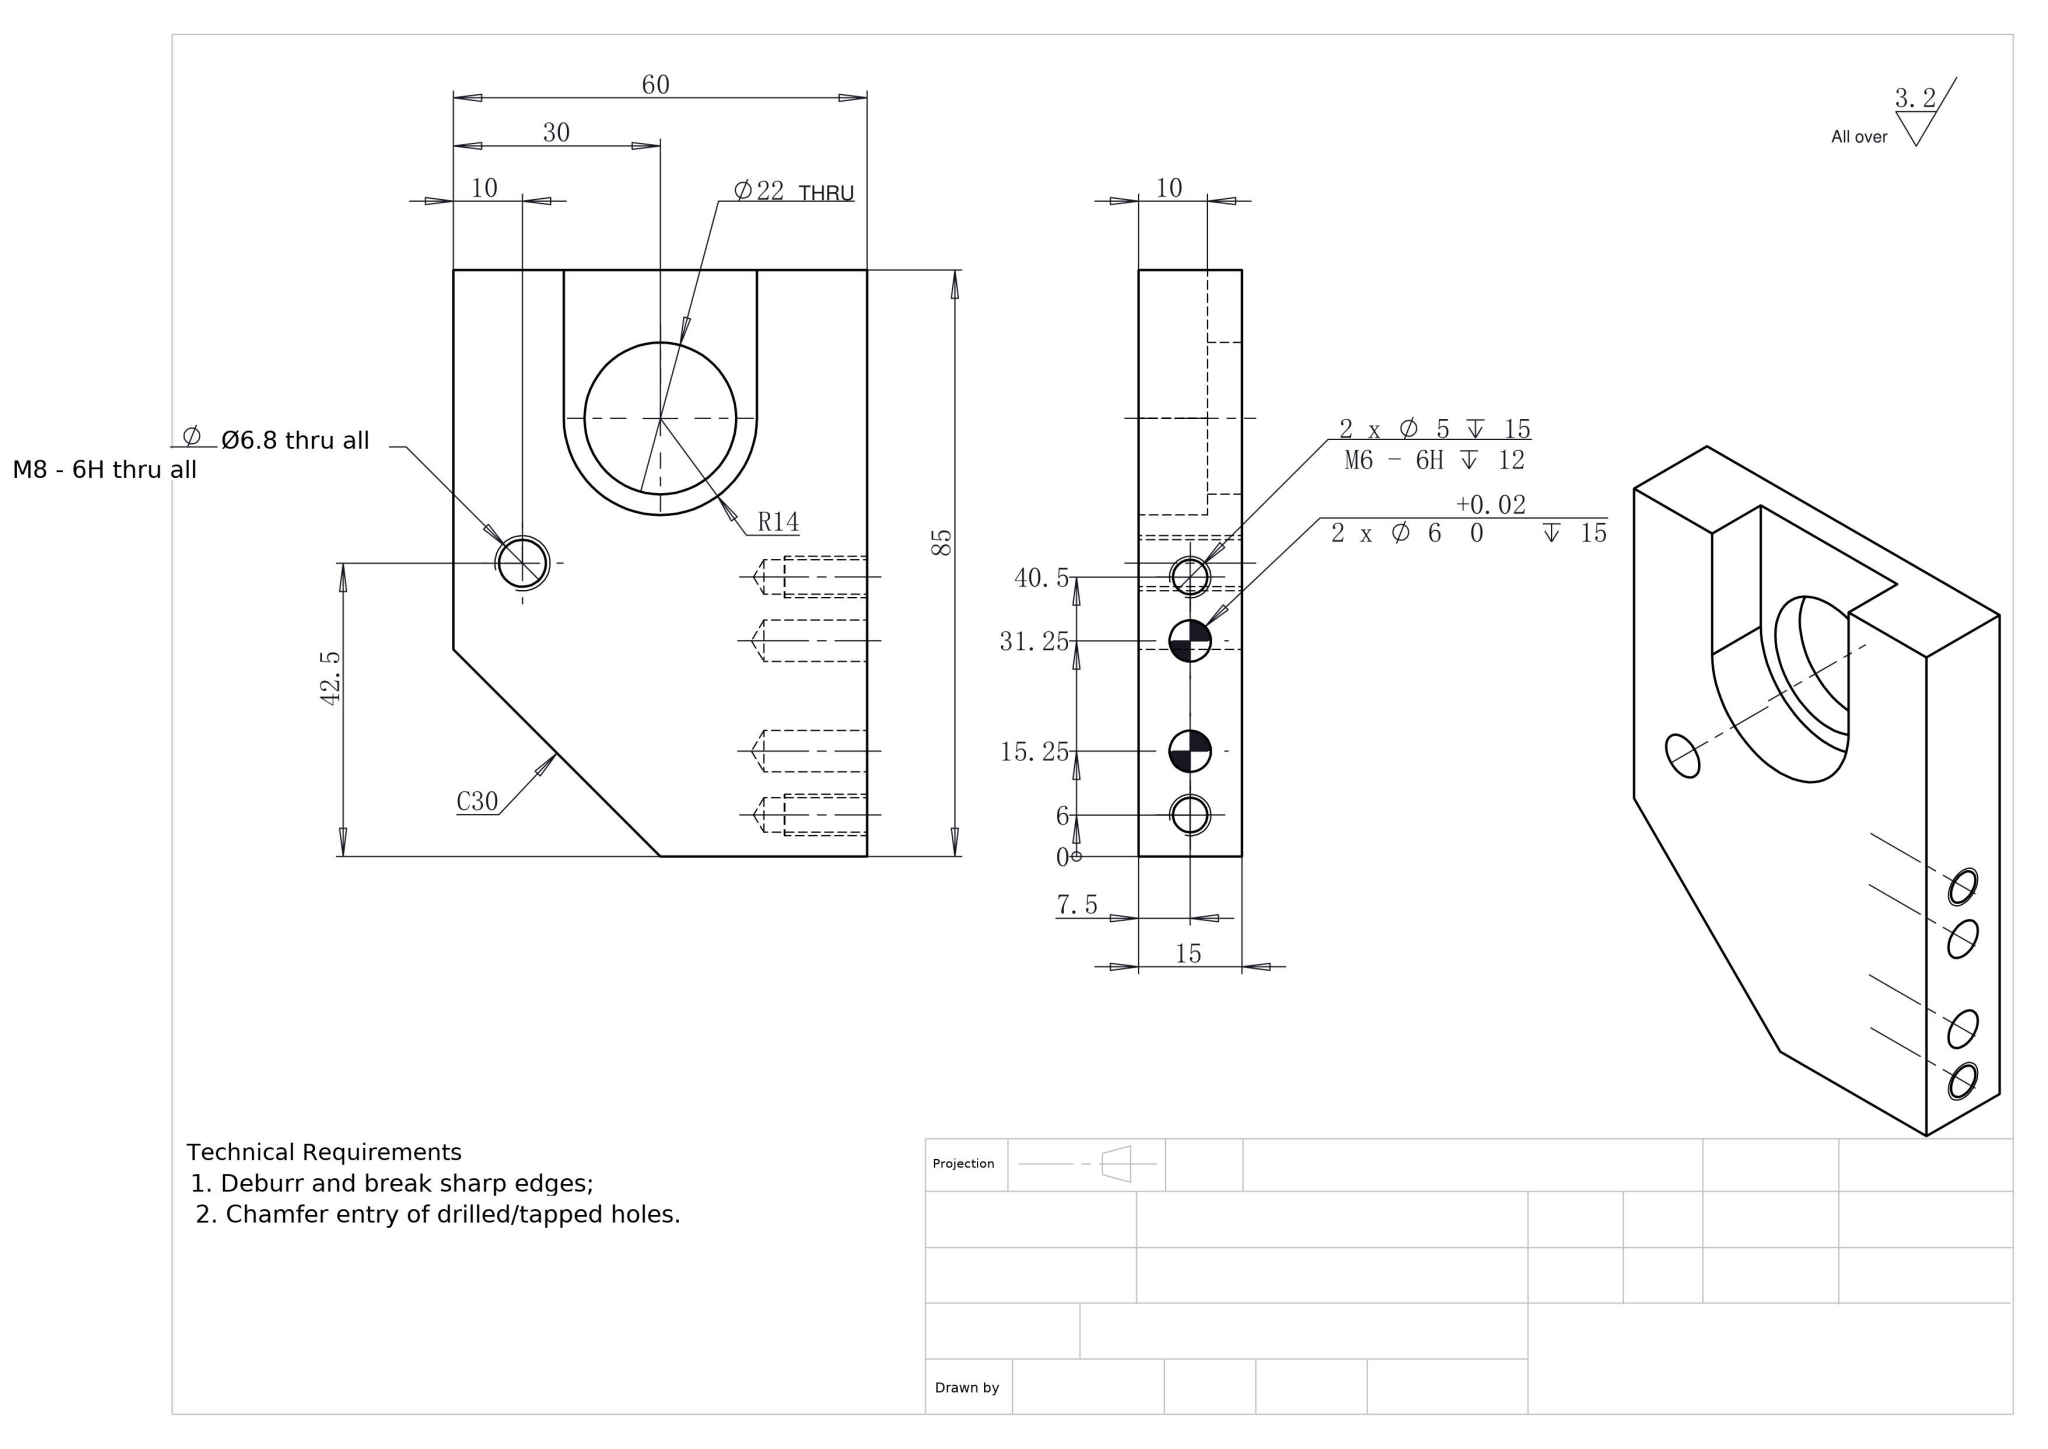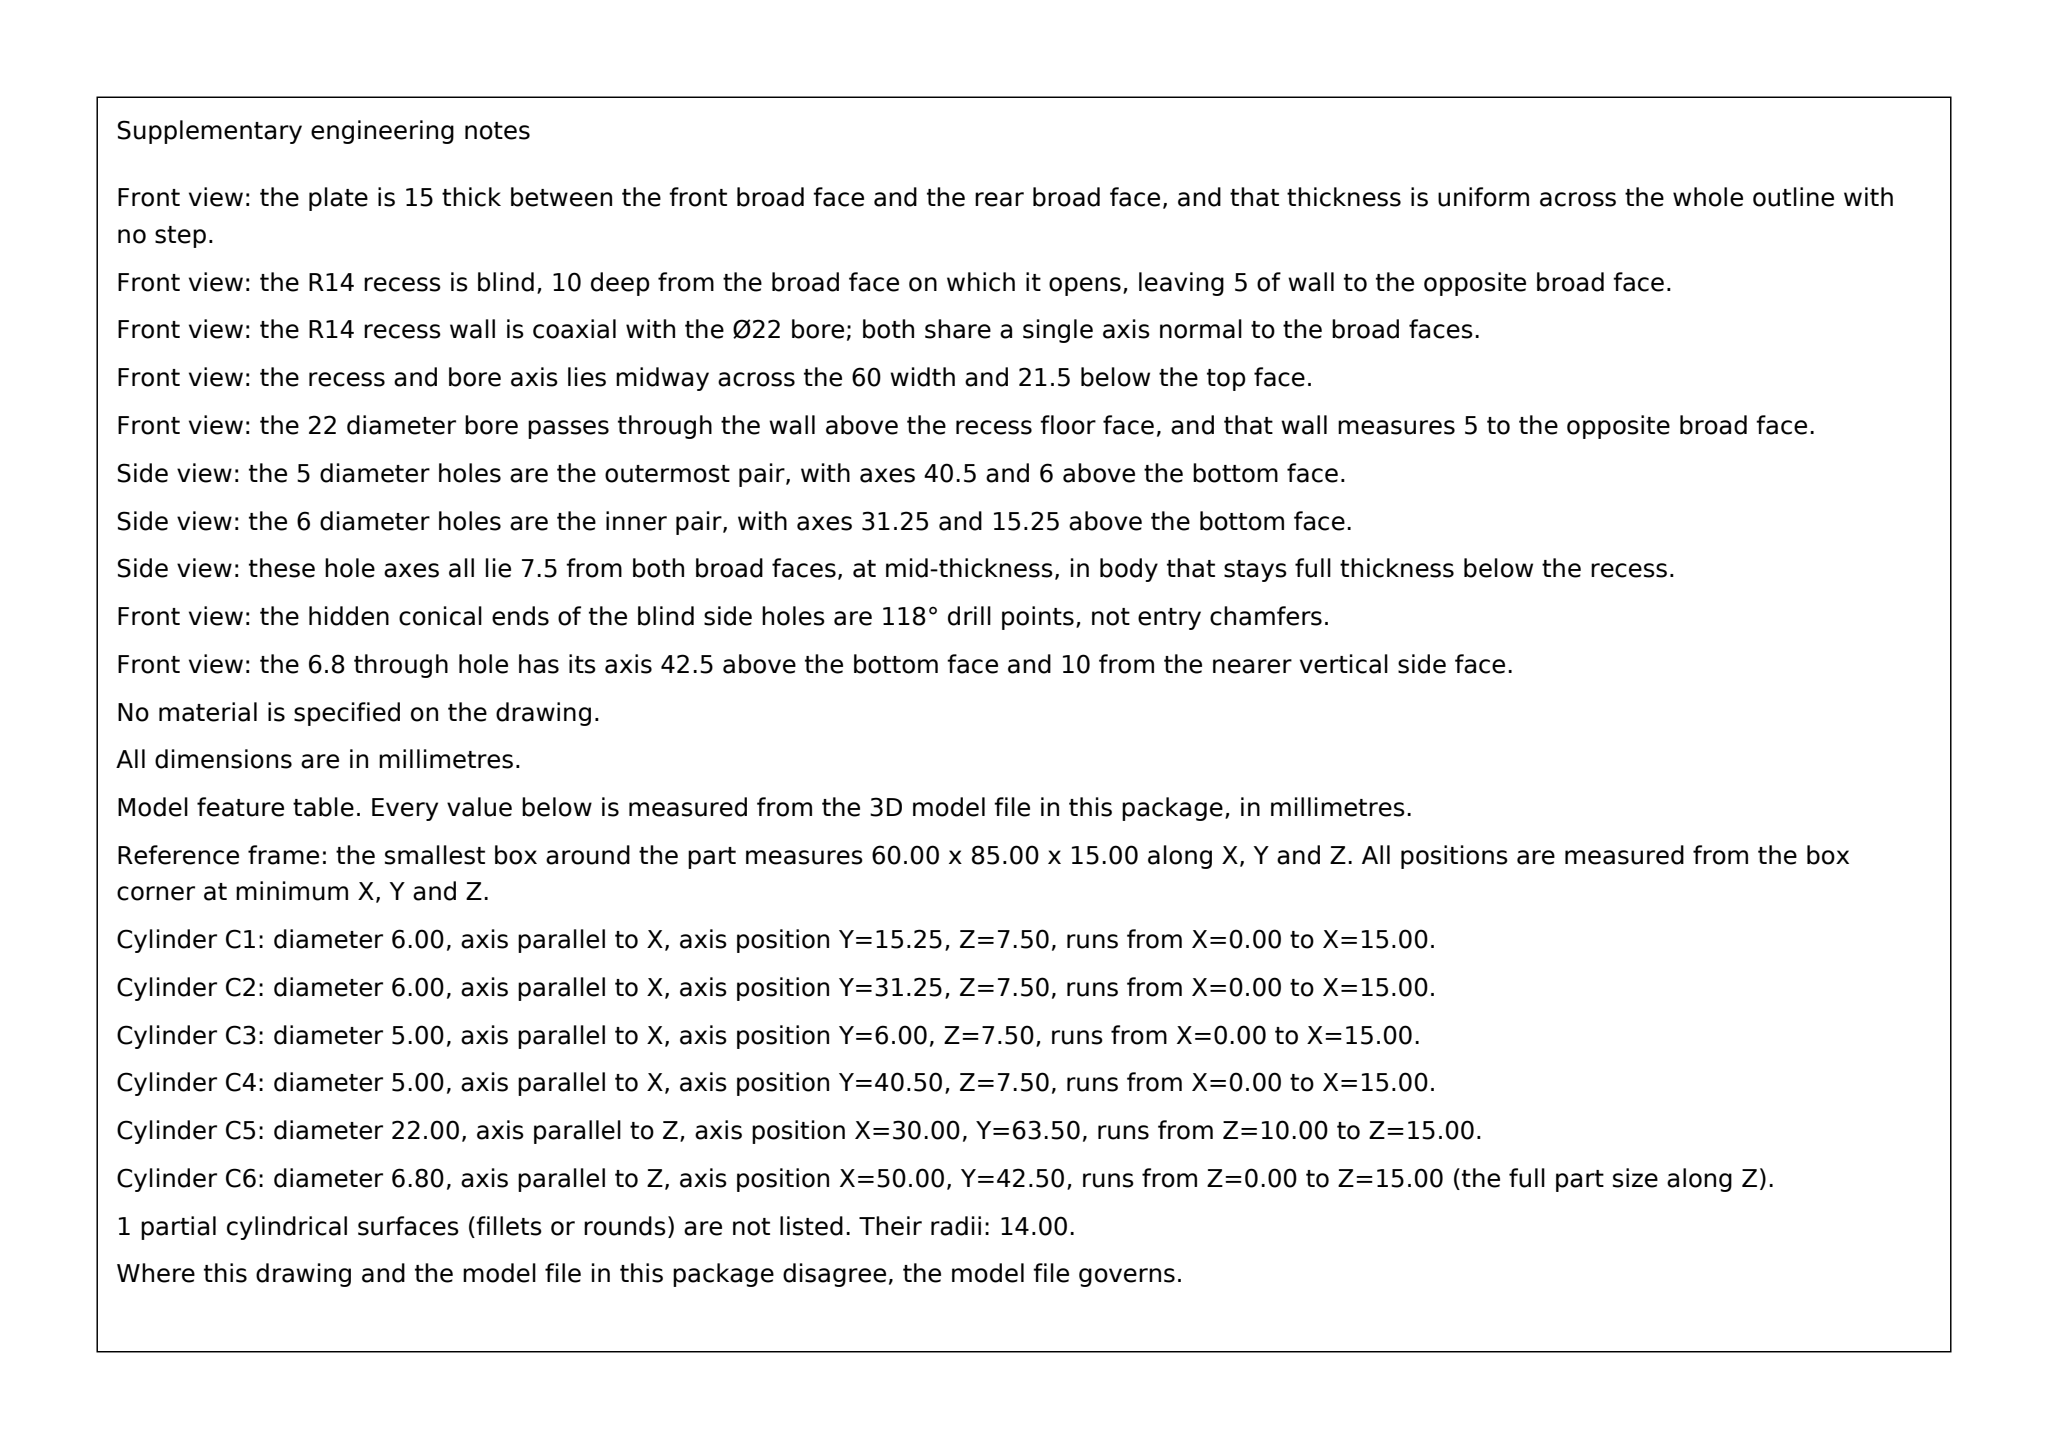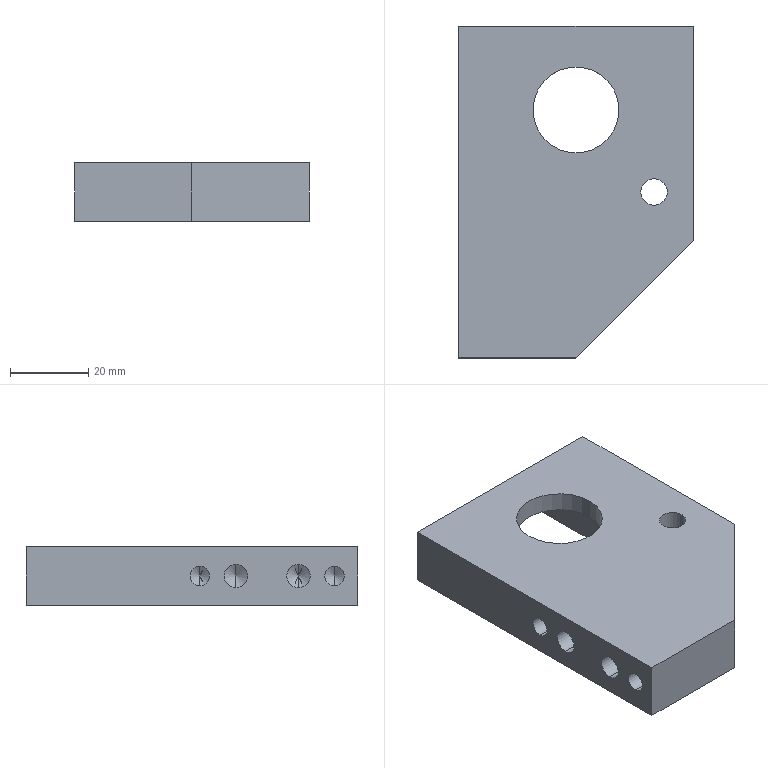Part | SolidWorks | mm | 1 solid | 31 faces | box 60 x 85 x 15 mm | volume 56715 mm3 | cylinder 13 | plane 10 | cone 8 | commonest cylinder face diameters 6 x4 5 x4 6.8 x2 22 x2 28 x1
Drawing notes:
Coaxial with Ø22: Ø28 counterbore/recess (R14) 10 deep from front face; Ø22 continues 5 thru remaining wall. | from the solid: cylinders[28.0,"z",[30.0,63.5],10.0] and cylinders[22.0,"z",[30.0,63.5],5.0]; bbox Z=15
All dimensions in millimetres (mm). | from the solid: STEP model facts stated in mm
build123d program:
from build123d import *

# Parameters (mm, degrees)
BOSS_EXTRUDE1_DEPTH          = 15
SKETCH2_R                    = 11
CUT_EXTRUDE1_DEPTH           = 106.119
CUT_EXTRUDE2_DEPTH           = 10
M8_TAPPED_HOLE1_D            = 6.8
M6_TAPPED_HOLE1_D            = 5
M6_TAPPED_HOLE1_DEPTH        = 15
M6_TAPPED_HOLE1_TIP          = 1.502
F_6_0_6_DIAMETER_HOLE1_D     = 6
F_6_0_6_DIAMETER_HOLE1_DEPTH = 15
F_6_0_6_DIAMETER_HOLE1_TIP   = 1.803


with BuildPart() as part:
    # Sketch1 → Boss-Extrude1 (new body)
    with BuildSketch(Plane.XY):
        Polygon((0, 0), (30, 0), (60, 30), (60, 85), (0, 85), align=None)
    extrude(amount=BOSS_EXTRUDE1_DEPTH)

    # Sketch2 → Cut-Extrude1 (cut, through all)
    with BuildSketch(Plane.XY.offset(15)):
        with Locations((30, 63.5)):
            Circle(SKETCH2_R)
    extrude(amount=-CUT_EXTRUDE1_DEPTH, mode=Mode.SUBTRACT)

    # Sketch3 → Cut-Extrude2 (cut)
    with BuildSketch(Plane(origin=(0, 0, 0), x_dir=(-1, 0, 0), z_dir=(0, 0, -1))):
        with BuildLine():
            Line((-44, 63.5), (-44, 85))
            ThreePointArc((-44, 85), (-30, 99), (-16, 85))
            Line((-16, 85), (-16, 63.5))
            ThreePointArc((-16, 63.5), (-30, 49.5), (-44, 63.5))
        make_face()
    extrude(amount=-CUT_EXTRUDE2_DEPTH, mode=Mode.SUBTRACT)

    # M8 Tapped Hole1 (through all)
    with Locations(Plane.XY.offset(15)):
        with Locations((50, 42.5)):
            Hole(M8_TAPPED_HOLE1_D / 2)

    # M6 Tapped Hole1
    with Locations(Plane.ZY):
        with Locations((7.5, 6), (7.5, 40.5)):
            Hole(M6_TAPPED_HOLE1_D / 2, depth=M6_TAPPED_HOLE1_DEPTH)
            with Locations((0, 0, -(M6_TAPPED_HOLE1_DEPTH + M6_TAPPED_HOLE1_TIP / 2))):  # 118° drill point
                Cone(0, M6_TAPPED_HOLE1_D / 2, M6_TAPPED_HOLE1_TIP, mode=Mode.SUBTRACT)

    # 6.0 _6_ Diameter Hole1
    with Locations(Plane.ZY):
        with Locations((7.5, 31.25), (7.5, 15.25)):
            Hole(F_6_0_6_DIAMETER_HOLE1_D / 2, depth=F_6_0_6_DIAMETER_HOLE1_DEPTH)
            with Locations((0, 0, -(F_6_0_6_DIAMETER_HOLE1_DEPTH + F_6_0_6_DIAMETER_HOLE1_TIP / 2))):  # 118° drill point
                Cone(0, F_6_0_6_DIAMETER_HOLE1_D / 2, F_6_0_6_DIAMETER_HOLE1_TIP, mode=Mode.SUBTRACT)


solid = part.part
STEP:
#1=CARTESIAN_POINT('',(15.,31.25,4.5));
#2=VERTEX_POINT('',#1);
#3=CARTESIAN_POINT('',(15.,31.25,10.5));
#4=VERTEX_POINT('',#3);
#5=CARTESIAN_POINT('',(15.,31.25,7.5));
#6=DIRECTION('',(-1.,0.,0.));
#7=DIRECTION('',(0.,0.,1.));
#8=AXIS2_PLACEMENT_3D('',#5,#6,#7);
#9=CIRCLE('',#8,3.);
#10=EDGE_CURVE('',#2,#4,#9,.T.);
#11=ORIENTED_EDGE('',*,*,#10,.F.);
#12=CARTESIAN_POINT('',(0.,31.25,4.5));
#13=VERTEX_POINT('',#12);
#14=CARTESIAN_POINT('',(0.,31.25,4.5));
#15=DIRECTION('',(-1.,0.,0.));
#16=VECTOR('',#15,1000.);
#17=LINE('',#14,#16);
#18=EDGE_CURVE('',#2,#13,#17,.T.);
#19=ORIENTED_EDGE('',*,*,#18,.T.);
#20=CARTESIAN_POINT('',(0.,31.25,10.5));
#21=VERTEX_POINT('',#20);
#22=CARTESIAN_POINT('',(0.,31.25,7.5));
#23=DIRECTION('',(-1.,0.,0.));
#24=DIRECTION('',(0.,0.,1.));
#25=AXIS2_PLACEMENT_3D('',#22,#23,#24);
#26=CIRCLE('',#25,3.);
#27=EDGE_CURVE('',#13,#21,#26,.T.);
#28=ORIENTED_EDGE('',*,*,#27,.T.);
#29=CARTESIAN_POINT('',(0.,31.25,10.5));
#30=DIRECTION('',(-1.,0.,0.));
#31=VECTOR('',#30,1000.);
#32=LINE('',#29,#31);
#33=EDGE_CURVE('',#4,#21,#32,.T.);
#34=ORIENTED_EDGE('',*,*,#33,.F.);
#35=EDGE_LOOP('',(#11,#19,#28,#34));
#36=FACE_OUTER_BOUND('',#35,.T.);
#37=CARTESIAN_POINT('',(0.,31.25,7.5));
#38=DIRECTION('',(-1.,0.,0.));
#39=DIRECTION('',(0.,0.,1.));
#40=AXIS2_PLACEMENT_3D('',#37,#38,#39);
#41=CYLINDRICAL_SURFACE('',#40,3.);
#42=ADVANCED_FACE('',(#36),#41,.F.);
#43=CARTESIAN_POINT('',(16.803,31.25,7.5));
#44=VERTEX_POINT('',#43);
#45=CARTESIAN_POINT('',(15.,31.25,10.5));
#46=DIRECTION('',(-0.515,0.,0.8572));
#47=VECTOR('',#46,1000.);
#48=LINE('',#45,#47);
#49=EDGE_CURVE('',#44,#4,#48,.T.);
#50=ORIENTED_EDGE('',*,*,#49,.F.);
#51=CARTESIAN_POINT('',(15.,31.25,4.5));
#52=DIRECTION('',(-0.515,0.,-0.8572));
#53=VECTOR('',#52,1000.);
#54=LINE('',#51,#53);
#55=EDGE_CURVE('',#44,#2,#54,.T.);
#56=ORIENTED_EDGE('',*,*,#55,.T.);
#57=ORIENTED_EDGE('',*,*,#10,.T.);
#58=EDGE_LOOP('',(#50,#56,#57));
#59=FACE_OUTER_BOUND('',#58,.T.);
#60=CARTESIAN_POINT('',(15.,31.25,7.5));
#61=DIRECTION('',(-1.,0.,0.));
#62=DIRECTION('',(0.,0.,1.));
#63=AXIS2_PLACEMENT_3D('',#60,#61,#62);
#64=CONICAL_SURFACE('',#63,3.,1.03);
#65=ADVANCED_FACE('',(#59),#64,.F.);
#66=CARTESIAN_POINT('',(15.,15.25,4.5));
#67=VERTEX_POINT('',#66);
#68=CARTESIAN_POINT('',(15.,15.25,10.5));
#69=VERTEX_POINT('',#68);
#70=CARTESIAN_POINT('',(15.,15.25,7.5));
#71=DIRECTION('',(-1.,0.,0.));
#72=DIRECTION('',(0.,0.,1.));
#73=AXIS2_PLACEMENT_3D('',#70,#71,#72);
#74=CIRCLE('',#73,3.);
#75=EDGE_CURVE('',#67,#69,#74,.T.);
#76=ORIENTED_EDGE('',*,*,#75,.F.);
#77=CARTESIAN_POINT('',(0.,15.25,4.5));
#78=VERTEX_POINT('',#77);
#79=CARTESIAN_POINT('',(0.,15.25,4.5));
#80=DIRECTION('',(-1.,0.,0.));
#81=VECTOR('',#80,1000.);
#82=LINE('',#79,#81);
#83=EDGE_CURVE('',#67,#78,#82,.T.);
#84=ORIENTED_EDGE('',*,*,#83,.T.);
#85=CARTESIAN_POINT('',(0.,15.25,10.5));
#86=VERTEX_POINT('',#85);
#87=CARTESIAN_POINT('',(0.,15.25,7.5));
#88=DIRECTION('',(-1.,0.,0.));
#89=DIRECTION('',(0.,0.,1.));
#90=AXIS2_PLACEMENT_3D('',#87,#88,#89);
#91=CIRCLE('',#90,3.);
#92=EDGE_CURVE('',#78,#86,#91,.T.);
#93=ORIENTED_EDGE('',*,*,#92,.T.);
#94=CARTESIAN_POINT('',(0.,15.25,10.5));
#95=DIRECTION('',(-1.,0.,0.));
#96=VECTOR('',#95,1000.);
#97=LINE('',#94,#96);
#98=EDGE_CURVE('',#69,#86,#97,.T.);
#99=ORIENTED_EDGE('',*,*,#98,.F.);
#100=EDGE_LOOP('',(#76,#84,#93,#99));
#101=FACE_OUTER_BOUND('',#100,.T.);
#102=CARTESIAN_POINT('',(0.,15.25,7.5));
#103=DIRECTION('',(-1.,0.,0.));
#104=DIRECTION('',(0.,0.,1.));
#105=AXIS2_PLACEMENT_3D('',#102,#103,#104);
#106=CYLINDRICAL_SURFACE('',#105,3.);
#107=ADVANCED_FACE('',(#101),#106,.F.);
#108=CARTESIAN_POINT('',(16.803,15.25,7.5));
#109=VERTEX_POINT('',#108);
#110=CARTESIAN_POINT('',(15.,15.25,10.5));
#111=DIRECTION('',(-0.515,0.,0.8572));
#112=VECTOR('',#111,1000.);
#113=LINE('',#110,#112);
#114=EDGE_CURVE('',#109,#69,#113,.T.);
#115=ORIENTED_EDGE('',*,*,#114,.F.);
#116=CARTESIAN_POINT('',(15.,15.25,4.5));
#117=DIRECTION('',(-0.515,0.,-0.8572));
#118=VECTOR('',#117,1000.);
#119=LINE('',#116,#118);
#120=EDGE_CURVE('',#109,#67,#119,.T.);
#121=ORIENTED_EDGE('',*,*,#120,.T.);
#122=ORIENTED_EDGE('',*,*,#75,.T.);
#123=EDGE_LOOP('',(#115,#121,#122));
#124=FACE_OUTER_BOUND('',#123,.T.);
#125=CARTESIAN_POINT('',(15.,15.25,7.5));
#126=DIRECTION('',(-1.,0.,0.));
#127=DIRECTION('',(0.,0.,1.));
#128=AXIS2_PLACEMENT_3D('',#125,#126,#127);
#129=CONICAL_SURFACE('',#128,3.,1.03);
#130=ADVANCED_FACE('',(#124),#129,.F.);
#131=CARTESIAN_POINT('',(15.,6.,5.));
#132=VERTEX_POINT('',#131);
#133=CARTESIAN_POINT('',(15.,6.,10.));
#134=VERTEX_POINT('',#133);
#135=CARTESIAN_POINT('',(15.,6.,7.5));
#136=DIRECTION('',(-1.,0.,0.));
#137=DIRECTION('',(0.,0.,1.));
#138=AXIS2_PLACEMENT_3D('',#135,#136,#137);
#139=CIRCLE('',#138,2.5);
#140=EDGE_CURVE('',#132,#134,#139,.T.);
#141=ORIENTED_EDGE('',*,*,#140,.F.);
#142=CARTESIAN_POINT('',(0.,6.,5.));
#143=VERTEX_POINT('',#142);
#144=CARTESIAN_POINT('',(0.,6.,5.));
#145=DIRECTION('',(-1.,0.,0.));
#146=VECTOR('',#145,1000.);
#147=LINE('',#144,#146);
#148=EDGE_CURVE('',#132,#143,#147,.T.);
#149=ORIENTED_EDGE('',*,*,#148,.T.);
#150=CARTESIAN_POINT('',(0.,6.,10.));
#151=VERTEX_POINT('',#150);
#152=CARTESIAN_POINT('',(0.,6.,7.5));
#153=DIRECTION('',(-1.,0.,0.));
#154=DIRECTION('',(0.,0.,1.));
#155=AXIS2_PLACEMENT_3D('',#152,#153,#154);
#156=CIRCLE('',#155,2.5);
#157=EDGE_CURVE('',#143,#151,#156,.T.);
#158=ORIENTED_EDGE('',*,*,#157,.T.);
#159=CARTESIAN_POINT('',(0.,6.,10.));
#160=DIRECTION('',(-1.,0.,0.));
#161=VECTOR('',#160,1000.);
#162=LINE('',#159,#161);
#163=EDGE_CURVE('',#134,#151,#162,.T.);
#164=ORIENTED_EDGE('',*,*,#163,.F.);
#165=EDGE_LOOP('',(#141,#149,#158,#164));
#166=FACE_OUTER_BOUND('',#165,.T.);
#167=CARTESIAN_POINT('',(0.,6.,7.5));
#168=DIRECTION('',(-1.,0.,0.));
#169=DIRECTION('',(0.,0.,1.));
#170=AXIS2_PLACEMENT_3D('',#167,#168,#169);
#171=CYLINDRICAL_SURFACE('',#170,2.5);
#172=ADVANCED_FACE('',(#166),#171,.F.);
#173=CARTESIAN_POINT('',(16.502,6.,7.5));
#174=VERTEX_POINT('',#173);
#175=CARTESIAN_POINT('',(15.,6.,10.));
#176=DIRECTION('',(-0.515,0.,0.8572));
#177=VECTOR('',#176,1000.);
#178=LINE('',#175,#177);
#179=EDGE_CURVE('',#174,#134,#178,.T.);
#180=ORIENTED_EDGE('',*,*,#179,.F.);
#181=CARTESIAN_POINT('',(15.,6.,5.));
#182=DIRECTION('',(-0.515,0.,-0.8572));
#183=VECTOR('',#182,1000.);
#184=LINE('',#181,#183);
#185=EDGE_CURVE('',#174,#132,#184,.T.);
#186=ORIENTED_EDGE('',*,*,#185,.T.);
#187=ORIENTED_EDGE('',*,*,#140,.T.);
#188=EDGE_LOOP('',(#180,#186,#187));
#189=FACE_OUTER_BOUND('',#188,.T.);
#190=CARTESIAN_POINT('',(15.,6.,7.5));
#191=DIRECTION('',(-1.,0.,0.));
#192=DIRECTION('',(0.,0.,1.));
#193=AXIS2_PLACEMENT_3D('',#190,#191,#192);
#194=CONICAL_SURFACE('',#193,2.5,1.03);
#195=ADVANCED_FACE('',(#189),#194,.F.);
#196=CARTESIAN_POINT('',(15.,40.5,5.));
#197=VERTEX_POINT('',#196);
#198=CARTESIAN_POINT('',(15.,40.5,10.));
#199=VERTEX_POINT('',#198);
#200=CARTESIAN_POINT('',(15.,40.5,7.5));
#201=DIRECTION('',(-1.,0.,0.));
#202=DIRECTION('',(0.,0.,1.));
#203=AXIS2_PLACEMENT_3D('',#200,#201,#202);
#204=CIRCLE('',#203,2.5);
#205=EDGE_CURVE('',#197,#199,#204,.T.);
#206=ORIENTED_EDGE('',*,*,#205,.F.);
#207=CARTESIAN_POINT('',(0.,40.5,5.));
#208=VERTEX_POINT('',#207);
#209=CARTESIAN_POINT('',(0.,40.5,5.));
#210=DIRECTION('',(-1.,0.,0.));
#211=VECTOR('',#210,1000.);
#212=LINE('',#209,#211);
#213=EDGE_CURVE('',#197,#208,#212,.T.);
#214=ORIENTED_EDGE('',*,*,#213,.T.);
#215=CARTESIAN_POINT('',(0.,40.5,10.));
#216=VERTEX_POINT('',#215);
#217=CARTESIAN_POINT('',(0.,40.5,7.5));
#218=DIRECTION('',(-1.,0.,0.));
#219=DIRECTION('',(0.,0.,1.));
#220=AXIS2_PLACEMENT_3D('',#217,#218,#219);
#221=CIRCLE('',#220,2.5);
#222=EDGE_CURVE('',#208,#216,#221,.T.);
#223=ORIENTED_EDGE('',*,*,#222,.T.);
#224=CARTESIAN_POINT('',(0.,40.5,10.));
#225=DIRECTION('',(-1.,0.,0.));
#226=VECTOR('',#225,1000.);
#227=LINE('',#224,#226);
#228=EDGE_CURVE('',#199,#216,#227,.T.);
#229=ORIENTED_EDGE('',*,*,#228,.F.);
#230=EDGE_LOOP('',(#206,#214,#223,#229));
#231=FACE_OUTER_BOUND('',#230,.T.);
#232=CARTESIAN_POINT('',(0.,40.5,7.5));
#233=DIRECTION('',(-1.,0.,0.));
#234=DIRECTION('',(0.,0.,1.));
#235=AXIS2_PLACEMENT_3D('',#232,#233,#234);
#236=CYLINDRICAL_SURFACE('',#235,2.5);
#237=ADVANCED_FACE('',(#231),#236,.F.);
#238=CARTESIAN_POINT('',(16.502,40.5,7.5));
#239=VERTEX_POINT('',#238);
#240=CARTESIAN_POINT('',(15.,40.5,10.));
#241=DIRECTION('',(-0.515,0.,0.8572));
#242=VECTOR('',#241,1000.);
#243=LINE('',#240,#242);
#244=EDGE_CURVE('',#239,#199,#243,.T.);
#245=ORIENTED_EDGE('',*,*,#244,.F.);
#246=CARTESIAN_POINT('',(15.,40.5,5.));
#247=DIRECTION('',(-0.515,0.,-0.8572));
#248=VECTOR('',#247,1000.);
#249=LINE('',#246,#248);
#250=EDGE_CURVE('',#239,#197,#249,.T.);
#251=ORIENTED_EDGE('',*,*,#250,.T.);
#252=ORIENTED_EDGE('',*,*,#205,.T.);
#253=EDGE_LOOP('',(#245,#251,#252));
#254=FACE_OUTER_BOUND('',#253,.T.);
#255=CARTESIAN_POINT('',(15.,40.5,7.5));
#256=DIRECTION('',(-1.,0.,0.));
#257=DIRECTION('',(0.,0.,1.));
#258=AXIS2_PLACEMENT_3D('',#255,#256,#257);
#259=CONICAL_SURFACE('',#258,2.5,1.03);
#260=ADVANCED_FACE('',(#254),#259,.F.);
#261=CARTESIAN_POINT('',(46.6,42.5,0.));
#262=VERTEX_POINT('',#261);
#263=CARTESIAN_POINT('',(53.4,42.5,0.));
#264=VERTEX_POINT('',#263);
#265=CARTESIAN_POINT('',(50.,42.5,0.));
#266=DIRECTION('',(0.,0.,1.));
#267=DIRECTION('',(1.,0.,0.));
#268=AXIS2_PLACEMENT_3D('',#265,#266,#267);
#269=CIRCLE('',#268,3.4);
#270=EDGE_CURVE('',#262,#264,#269,.T.);
#271=ORIENTED_EDGE('',*,*,#270,.F.);
#272=CARTESIAN_POINT('',(46.6,42.5,15.));
#273=VERTEX_POINT('',#272);
#274=CARTESIAN_POINT('',(46.6,42.5,15.));
#275=DIRECTION('',(0.,0.,1.));
#276=VECTOR('',#275,1000.);
#277=LINE('',#274,#276);
#278=EDGE_CURVE('',#262,#273,#277,.T.);
#279=ORIENTED_EDGE('',*,*,#278,.T.);
#280=CARTESIAN_POINT('',(53.4,42.5,15.));
#281=VERTEX_POINT('',#280);
#282=CARTESIAN_POINT('',(50.,42.5,15.));
#283=DIRECTION('',(0.,0.,1.));
#284=DIRECTION('',(1.,0.,0.));
#285=AXIS2_PLACEMENT_3D('',#282,#283,#284);
#286=CIRCLE('',#285,3.4);
#287=EDGE_CURVE('',#273,#281,#286,.T.);
#288=ORIENTED_EDGE('',*,*,#287,.T.);
#289=CARTESIAN_POINT('',(53.4,42.5,15.));
#290=DIRECTION('',(0.,0.,1.));
#291=VECTOR('',#290,1000.);
#292=LINE('',#289,#291);
#293=EDGE_CURVE('',#264,#281,#292,.T.);
#294=ORIENTED_EDGE('',*,*,#293,.F.);
#295=EDGE_LOOP('',(#271,#279,#288,#294));
#296=FACE_OUTER_BOUND('',#295,.T.);
#297=CARTESIAN_POINT('',(50.,42.5,15.));
#298=DIRECTION('',(0.,0.,1.));
#299=DIRECTION('',(1.,0.,0.));
#300=AXIS2_PLACEMENT_3D('',#297,#298,#299);
#301=CYLINDRICAL_SURFACE('',#300,3.4);
#302=ADVANCED_FACE('',(#296),#301,.F.);
#303=CARTESIAN_POINT('',(19.,63.5,10.));
#304=VERTEX_POINT('',#303);
#305=CARTESIAN_POINT('',(41.,63.5,10.));
#306=VERTEX_POINT('',#305);
#307=CARTESIAN_POINT('',(30.,63.5,10.));
#308=DIRECTION('',(0.,0.,1.));
#309=DIRECTION('',(-1.,0.,0.));
#310=AXIS2_PLACEMENT_3D('',#307,#308,#309);
#311=CIRCLE('',#310,11.);
#312=EDGE_CURVE('',#304,#306,#311,.T.);
#313=ORIENTED_EDGE('',*,*,#312,.F.);
#314=CARTESIAN_POINT('',(19.,63.5,15.));
#315=VERTEX_POINT('',#314);
#316=CARTESIAN_POINT('',(19.,63.5,0.));
#317=DIRECTION('',(0.,0.,1.));
#318=VECTOR('',#317,1000.);
#319=LINE('',#316,#318);
#320=EDGE_CURVE('',#304,#315,#319,.T.);
#321=ORIENTED_EDGE('',*,*,#320,.T.);
#322=CARTESIAN_POINT('',(41.,63.5,15.));
#323=VERTEX_POINT('',#322);
#324=CARTESIAN_POINT('',(30.,63.5,15.));
#325=DIRECTION('',(0.,0.,1.));
#326=DIRECTION('',(1.,0.,0.));
#327=AXIS2_PLACEMENT_3D('',#324,#325,#326);
#328=CIRCLE('',#327,11.);
#329=EDGE_CURVE('',#315,#323,#328,.T.);
#330=ORIENTED_EDGE('',*,*,#329,.T.);
#331=CARTESIAN_POINT('',(41.,63.5,0.));
#332=DIRECTION('',(0.,0.,1.));
#333=VECTOR('',#332,1000.);
#334=LINE('',#331,#333);
#335=EDGE_CURVE('',#306,#323,#334,.T.);
#336=ORIENTED_EDGE('',*,*,#335,.F.);
#337=EDGE_LOOP('',(#313,#321,#330,#336));
#338=FACE_OUTER_BOUND('',#337,.T.);
#339=CARTESIAN_POINT('',(30.,63.5,0.));
#340=DIRECTION('',(0.,0.,1.));
#341=DIRECTION('',(1.,0.,0.));
#342=AXIS2_PLACEMENT_3D('',#339,#340,#341);
#343=CYLINDRICAL_SURFACE('',#342,11.);
#344=ADVANCED_FACE('',(#338),#343,.F.);
#345=ORIENTED_EDGE('',*,*,#320,.F.);
#346=CARTESIAN_POINT('',(30.,63.5,10.));
#347=DIRECTION('',(0.,0.,1.));
#348=DIRECTION('',(-1.,0.,0.));
#349=AXIS2_PLACEMENT_3D('',#346,#347,#348);
#350=CIRCLE('',#349,11.);
#351=EDGE_CURVE('',#306,#304,#350,.T.);
#352=ORIENTED_EDGE('',*,*,#351,.F.);
#353=ORIENTED_EDGE('',*,*,#335,.T.);
#354=CARTESIAN_POINT('',(30.,63.5,15.));
#355=DIRECTION('',(0.,0.,1.));
#356=DIRECTION('',(1.,0.,0.));
#357=AXIS2_PLACEMENT_3D('',#354,#355,#356);
#358=CIRCLE('',#357,11.);
#359=EDGE_CURVE('',#323,#315,#358,.T.);
#360=ORIENTED_EDGE('',*,*,#359,.T.);
#361=EDGE_LOOP('',(#345,#352,#353,#360));
#362=FACE_OUTER_BOUND('',#361,.T.);
#363=CARTESIAN_POINT('',(30.,63.5,0.));
#364=DIRECTION('',(0.,0.,1.));
#365=DIRECTION('',(1.,0.,0.));
#366=AXIS2_PLACEMENT_3D('',#363,#364,#365);
#367=CYLINDRICAL_SURFACE('',#366,11.);
#368=ADVANCED_FACE('',(#362),#367,.F.);
#369=CARTESIAN_POINT('',(44.,85.,10.));
#370=VERTEX_POINT('',#369);
#371=CARTESIAN_POINT('',(44.,85.,0.));
#372=VERTEX_POINT('',#371);
#373=CARTESIAN_POINT('',(44.,85.,10.));
#374=DIRECTION('',(0.,0.,-1.));
#375=VECTOR('',#374,1000.);
#376=LINE('',#373,#375);
#377=EDGE_CURVE('',#370,#372,#376,.T.);
#378=ORIENTED_EDGE('',*,*,#377,.F.);
#379=CARTESIAN_POINT('',(16.,85.,10.));
#380=VERTEX_POINT('',#379);
#381=CARTESIAN_POINT('',(0.,85.,10.));
#382=DIRECTION('',(-1.,0.,0.));
#383=VECTOR('',#382,1000.);
#384=LINE('',#381,#383);
#385=EDGE_CURVE('',#370,#380,#384,.T.);
#386=ORIENTED_EDGE('',*,*,#385,.T.);
#387=CARTESIAN_POINT('',(16.,85.,0.));
#388=VERTEX_POINT('',#387);
#389=CARTESIAN_POINT('',(16.,85.,10.));
#390=DIRECTION('',(0.,0.,-1.));
#391=VECTOR('',#390,1000.);
#392=LINE('',#389,#391);
#393=EDGE_CURVE('',#380,#388,#392,.T.);
#394=ORIENTED_EDGE('',*,*,#393,.T.);
#395=CARTESIAN_POINT('',(0.,85.,0.));
#396=VERTEX_POINT('',#395);
#397=CARTESIAN_POINT('',(0.,85.,0.));
#398=DIRECTION('',(1.,0.,0.));
#399=VECTOR('',#398,1000.);
#400=LINE('',#397,#399);
#401=EDGE_CURVE('',#396,#388,#400,.T.);
#402=ORIENTED_EDGE('',*,*,#401,.F.);
#403=CARTESIAN_POINT('',(0.,85.,15.));
#404=VERTEX_POINT('',#403);
#405=CARTESIAN_POINT('',(0.,85.,15.));
#406=DIRECTION('',(0.,0.,-1.));
#407=VECTOR('',#406,1000.);
#408=LINE('',#405,#407);
#409=EDGE_CURVE('',#404,#396,#408,.T.);
#410=ORIENTED_EDGE('',*,*,#409,.F.);
#411=CARTESIAN_POINT('',(60.,85.,15.));
#412=VERTEX_POINT('',#411);
#413=CARTESIAN_POINT('',(0.,85.,15.));
#414=DIRECTION('',(1.,0.,0.));
#415=VECTOR('',#414,1000.);
#416=LINE('',#413,#415);
#417=EDGE_CURVE('',#404,#412,#416,.T.);
#418=ORIENTED_EDGE('',*,*,#417,.T.);
#419=CARTESIAN_POINT('',(60.,85.,0.));
#420=VERTEX_POINT('',#419);
#421=CARTESIAN_POINT('',(60.,85.,15.));
#422=DIRECTION('',(0.,0.,-1.));
#423=VECTOR('',#422,1000.);
#424=LINE('',#421,#423);
#425=EDGE_CURVE('',#412,#420,#424,.T.);
#426=ORIENTED_EDGE('',*,*,#425,.T.);
#427=CARTESIAN_POINT('',(0.,85.,0.));
#428=DIRECTION('',(1.,0.,0.));
#429=VECTOR('',#428,1000.);
#430=LINE('',#427,#429);
#431=EDGE_CURVE('',#372,#420,#430,.T.);
#432=ORIENTED_EDGE('',*,*,#431,.F.);
#433=EDGE_LOOP('',(#378,#386,#394,#402,#410,#418,#426,#432));
#434=FACE_OUTER_BOUND('',#433,.T.);
#435=CARTESIAN_POINT('',(0.,85.,15.));
#436=DIRECTION('',(0.,1.,0.));
#437=DIRECTION('',(0.,0.,1.));
#438=AXIS2_PLACEMENT_3D('',#435,#436,#437);
#439=PLANE('',#438);
#440=ADVANCED_FACE('',(#434),#439,.T.);
#441=CARTESIAN_POINT('',(0.,31.25,7.5));
#442=DIRECTION('',(-1.,0.,0.));
#443=DIRECTION('',(0.,0.,1.));
#444=AXIS2_PLACEMENT_3D('',#441,#442,#443);
#445=CIRCLE('',#444,3.);
#446=EDGE_CURVE('',#21,#13,#445,.T.);
#447=ORIENTED_EDGE('',*,*,#446,.F.);
#448=ORIENTED_EDGE('',*,*,#27,.F.);
#449=EDGE_LOOP('',(#447,#448));
#450=FACE_BOUND('',#449,.T.);
#451=CARTESIAN_POINT('',(0.,15.25,7.5));
#452=DIRECTION('',(-1.,0.,0.));
#453=DIRECTION('',(0.,0.,1.));
#454=AXIS2_PLACEMENT_3D('',#451,#452,#453);
#455=CIRCLE('',#454,3.);
#456=EDGE_CURVE('',#86,#78,#455,.T.);
#457=ORIENTED_EDGE('',*,*,#456,.F.);
#458=ORIENTED_EDGE('',*,*,#92,.F.);
#459=EDGE_LOOP('',(#457,#458));
#460=FACE_BOUND('',#459,.T.);
#461=CARTESIAN_POINT('',(0.,6.,7.5));
#462=DIRECTION('',(-1.,0.,0.));
#463=DIRECTION('',(0.,0.,1.));
#464=AXIS2_PLACEMENT_3D('',#461,#462,#463);
#465=CIRCLE('',#464,2.5);
#466=EDGE_CURVE('',#151,#143,#465,.T.);
#467=ORIENTED_EDGE('',*,*,#466,.F.);
#468=ORIENTED_EDGE('',*,*,#157,.F.);
#469=EDGE_LOOP('',(#467,#468));
#470=FACE_BOUND('',#469,.T.);
#471=CARTESIAN_POINT('',(0.,40.5,7.5));
#472=DIRECTION('',(-1.,0.,0.));
#473=DIRECTION('',(0.,0.,1.));
#474=AXIS2_PLACEMENT_3D('',#471,#472,#473);
#475=CIRCLE('',#474,2.5);
#476=EDGE_CURVE('',#216,#208,#475,.T.);
#477=ORIENTED_EDGE('',*,*,#476,.F.);
#478=ORIENTED_EDGE('',*,*,#222,.F.);
#479=EDGE_LOOP('',(#477,#478));
#480=FACE_BOUND('',#479,.T.);
#481=CARTESIAN_POINT('',(0.,0.,0.));
#482=VERTEX_POINT('',#481);
#483=CARTESIAN_POINT('',(0.,85.,0.));
#484=DIRECTION('',(-0.,-1.,0.));
#485=VECTOR('',#484,1000.);
#486=LINE('',#483,#485);
#487=EDGE_CURVE('',#396,#482,#486,.T.);
#488=ORIENTED_EDGE('',*,*,#487,.T.);
#489=CARTESIAN_POINT('',(0.,0.,15.));
#490=VERTEX_POINT('',#489);
#491=CARTESIAN_POINT('',(0.,0.,15.));
#492=DIRECTION('',(0.,0.,-1.));
#493=VECTOR('',#492,1000.);
#494=LINE('',#491,#493);
#495=EDGE_CURVE('',#490,#482,#494,.T.);
#496=ORIENTED_EDGE('',*,*,#495,.F.);
#497=CARTESIAN_POINT('',(0.,85.,15.));
#498=DIRECTION('',(-0.,-1.,0.));
#499=VECTOR('',#498,1000.);
#500=LINE('',#497,#499);
#501=EDGE_CURVE('',#404,#490,#500,.T.);
#502=ORIENTED_EDGE('',*,*,#501,.F.);
#503=ORIENTED_EDGE('',*,*,#409,.T.);
#504=EDGE_LOOP('',(#488,#496,#502,#503));
#505=FACE_OUTER_BOUND('',#504,.T.);
#506=CARTESIAN_POINT('',(0.,85.,15.));
#507=DIRECTION('',(1.,-0.,0.));
#508=DIRECTION('',(0.,1.,0.));
#509=AXIS2_PLACEMENT_3D('',#506,#507,#508);
#510=PLANE('',#509);
#511=ADVANCED_FACE('',(#450,#460,#470,#480,#505),#510,.F.);
#512=CARTESIAN_POINT('',(30.,0.,0.));
#513=VERTEX_POINT('',#512);
#514=CARTESIAN_POINT('',(0.,0.,0.));
#515=DIRECTION('',(1.,0.,0.));
#516=VECTOR('',#515,1000.);
#517=LINE('',#514,#516);
#518=EDGE_CURVE('',#482,#513,#517,.T.);
#519=ORIENTED_EDGE('',*,*,#518,.T.);
#520=CARTESIAN_POINT('',(30.,0.,15.));
#521=VERTEX_POINT('',#520);
#522=CARTESIAN_POINT('',(30.,0.,15.));
#523=DIRECTION('',(0.,0.,-1.));
#524=VECTOR('',#523,1000.);
#525=LINE('',#522,#524);
#526=EDGE_CURVE('',#521,#513,#525,.T.);
#527=ORIENTED_EDGE('',*,*,#526,.F.);
#528=CARTESIAN_POINT('',(0.,0.,15.));
#529=DIRECTION('',(1.,0.,0.));
#530=VECTOR('',#529,1000.);
#531=LINE('',#528,#530);
#532=EDGE_CURVE('',#490,#521,#531,.T.);
#533=ORIENTED_EDGE('',*,*,#532,.F.);
#534=ORIENTED_EDGE('',*,*,#495,.T.);
#535=EDGE_LOOP('',(#519,#527,#533,#534));
#536=FACE_OUTER_BOUND('',#535,.T.);
#537=CARTESIAN_POINT('',(0.,0.,15.));
#538=DIRECTION('',(0.,1.,0.));
#539=DIRECTION('',(0.,0.,1.));
#540=AXIS2_PLACEMENT_3D('',#537,#538,#539);
#541=PLANE('',#540);
#542=ADVANCED_FACE('',(#536),#541,.F.);
#543=CARTESIAN_POINT('',(60.,30.,0.));
#544=VERTEX_POINT('',#543);
#545=CARTESIAN_POINT('',(30.,0.,0.));
#546=DIRECTION('',(0.7071,0.7071,0.));
#547=VECTOR('',#546,1000.);
#548=LINE('',#545,#547);
#549=EDGE_CURVE('',#513,#544,#548,.T.);
#550=ORIENTED_EDGE('',*,*,#549,.T.);
#551=CARTESIAN_POINT('',(60.,30.,15.));
#552=VERTEX_POINT('',#551);
#553=CARTESIAN_POINT('',(60.,30.,15.));
#554=DIRECTION('',(0.,0.,-1.));
#555=VECTOR('',#554,1000.);
#556=LINE('',#553,#555);
#557=EDGE_CURVE('',#552,#544,#556,.T.);
#558=ORIENTED_EDGE('',*,*,#557,.F.);
#559=CARTESIAN_POINT('',(30.,0.,15.));
#560=DIRECTION('',(0.7071,0.7071,0.));
#561=VECTOR('',#560,1000.);
#562=LINE('',#559,#561);
#563=EDGE_CURVE('',#521,#552,#562,.T.);
#564=ORIENTED_EDGE('',*,*,#563,.F.);
#565=ORIENTED_EDGE('',*,*,#526,.T.);
#566=EDGE_LOOP('',(#550,#558,#564,#565));
#567=FACE_OUTER_BOUND('',#566,.T.);
#568=CARTESIAN_POINT('',(30.,0.,15.));
#569=DIRECTION('',(-0.7071,0.7071,0.));
#570=DIRECTION('',(-0.7071,-0.7071,0.));
#571=AXIS2_PLACEMENT_3D('',#568,#569,#570);
#572=PLANE('',#571);
#573=ADVANCED_FACE('',(#567),#572,.F.);
#574=CARTESIAN_POINT('',(60.,85.,0.));
#575=DIRECTION('',(0.,-1.,0.));
#576=VECTOR('',#575,1000.);
#577=LINE('',#574,#576);
#578=EDGE_CURVE('',#420,#544,#577,.T.);
#579=ORIENTED_EDGE('',*,*,#578,.F.);
#580=ORIENTED_EDGE('',*,*,#425,.F.);
#581=CARTESIAN_POINT('',(60.,85.,15.));
#582=DIRECTION('',(0.,-1.,0.));
#583=VECTOR('',#582,1000.);
#584=LINE('',#581,#583);
#585=EDGE_CURVE('',#412,#552,#584,.T.);
#586=ORIENTED_EDGE('',*,*,#585,.T.);
#587=ORIENTED_EDGE('',*,*,#557,.T.);
#588=EDGE_LOOP('',(#579,#580,#586,#587));
#589=FACE_OUTER_BOUND('',#588,.T.);
#590=CARTESIAN_POINT('',(60.,85.,15.));
#591=DIRECTION('',(1.,0.,0.));
#592=DIRECTION('',(0.,0.,-1.));
#593=AXIS2_PLACEMENT_3D('',#590,#591,#592);
#594=PLANE('',#593);
#595=ADVANCED_FACE('',(#589),#594,.T.);
#596=CARTESIAN_POINT('',(50.,42.5,15.));
#597=DIRECTION('',(0.,0.,1.));
#598=DIRECTION('',(1.,0.,0.));
#599=AXIS2_PLACEMENT_3D('',#596,#597,#598);
#600=CIRCLE('',#599,3.4);
#601=EDGE_CURVE('',#281,#273,#600,.T.);
#602=ORIENTED_EDGE('',*,*,#601,.F.);
#603=ORIENTED_EDGE('',*,*,#287,.F.);
#604=EDGE_LOOP('',(#602,#603));
#605=FACE_BOUND('',#604,.T.);
#606=ORIENTED_EDGE('',*,*,#359,.F.);
#607=ORIENTED_EDGE('',*,*,#329,.F.);
#608=EDGE_LOOP('',(#606,#607));
#609=FACE_BOUND('',#608,.T.);
#610=ORIENTED_EDGE('',*,*,#417,.F.);
#611=ORIENTED_EDGE('',*,*,#501,.T.);
#612=ORIENTED_EDGE('',*,*,#532,.T.);
#613=ORIENTED_EDGE('',*,*,#563,.T.);
#614=ORIENTED_EDGE('',*,*,#585,.F.);
#615=EDGE_LOOP('',(#610,#611,#612,#613,#614));
#616=FACE_OUTER_BOUND('',#615,.T.);
#617=CARTESIAN_POINT('',(0.,0.,15.));
#618=DIRECTION('',(0.,0.,-1.));
#619=DIRECTION('',(-1.,0.,0.));
#620=AXIS2_PLACEMENT_3D('',#617,#618,#619);
#621=PLANE('',#620);
#622=ADVANCED_FACE('',(#605,#609,#616),#621,.F.);
#623=CARTESIAN_POINT('',(50.,42.5,0.));
#624=DIRECTION('',(0.,0.,1.));
#625=DIRECTION('',(1.,0.,0.));
#626=AXIS2_PLACEMENT_3D('',#623,#624,#625);
#627=CIRCLE('',#626,3.4);
#628=EDGE_CURVE('',#264,#262,#627,.T.);
#629=ORIENTED_EDGE('',*,*,#628,.T.);
#630=ORIENTED_EDGE('',*,*,#270,.T.);
#631=EDGE_LOOP('',(#629,#630));
#632=FACE_BOUND('',#631,.T.);
#633=CARTESIAN_POINT('',(44.,63.5,0.));
#634=VERTEX_POINT('',#633);
#635=CARTESIAN_POINT('',(44.,63.5,0.));
#636=DIRECTION('',(0.,-1.,0.));
#637=VECTOR('',#636,1000.);
#638=LINE('',#635,#637);
#639=EDGE_CURVE('',#372,#634,#638,.T.);
#640=ORIENTED_EDGE('',*,*,#639,.F.);
#641=ORIENTED_EDGE('',*,*,#431,.T.);
#642=ORIENTED_EDGE('',*,*,#578,.T.);
#643=ORIENTED_EDGE('',*,*,#549,.F.);
#644=ORIENTED_EDGE('',*,*,#518,.F.);
#645=ORIENTED_EDGE('',*,*,#487,.F.);
#646=ORIENTED_EDGE('',*,*,#401,.T.);
#647=CARTESIAN_POINT('',(16.,63.5,0.));
#648=VERTEX_POINT('',#647);
#649=CARTESIAN_POINT('',(16.,63.5,0.));
#650=DIRECTION('',(0.,1.,0.));
#651=VECTOR('',#650,1000.);
#652=LINE('',#649,#651);
#653=EDGE_CURVE('',#648,#388,#652,.T.);
#654=ORIENTED_EDGE('',*,*,#653,.F.);
#655=CARTESIAN_POINT('',(30.,63.5,0.));
#656=DIRECTION('',(0.,0.,-1.));
#657=DIRECTION('',(-1.,0.,0.));
#658=AXIS2_PLACEMENT_3D('',#655,#656,#657);
#659=CIRCLE('',#658,14.);
#660=EDGE_CURVE('',#634,#648,#659,.T.);
#661=ORIENTED_EDGE('',*,*,#660,.F.);
#662=EDGE_LOOP('',(#640,#641,#642,#643,#644,#645,#646,#654,#661));
#663=FACE_OUTER_BOUND('',#662,.T.);
#664=CARTESIAN_POINT('',(0.,0.,0.));
#665=DIRECTION('',(0.,0.,-1.));
#666=DIRECTION('',(-1.,0.,0.));
#667=AXIS2_PLACEMENT_3D('',#664,#665,#666);
#668=PLANE('',#667);
#669=ADVANCED_FACE('',(#632,#663),#668,.T.);
#670=CARTESIAN_POINT('',(44.,63.5,10.));
#671=VERTEX_POINT('',#670);
#672=CARTESIAN_POINT('',(44.,63.5,10.));
#673=DIRECTION('',(0.,-1.,0.));
#674=VECTOR('',#673,1000.);
#675=LINE('',#672,#674);
#676=EDGE_CURVE('',#370,#671,#675,.T.);
#677=ORIENTED_EDGE('',*,*,#676,.T.);
#678=CARTESIAN_POINT('',(16.,63.5,10.));
#679=VERTEX_POINT('',#678);
#680=CARTESIAN_POINT('',(30.,63.5,10.));
#681=DIRECTION('',(0.,0.,-1.));
#682=DIRECTION('',(-1.,0.,0.));
#683=AXIS2_PLACEMENT_3D('',#680,#681,#682);
#684=CIRCLE('',#683,14.);
#685=EDGE_CURVE('',#671,#679,#684,.T.);
#686=ORIENTED_EDGE('',*,*,#685,.T.);
#687=CARTESIAN_POINT('',(16.,63.5,10.));
#688=DIRECTION('',(0.,1.,0.));
#689=VECTOR('',#688,1000.);
#690=LINE('',#687,#689);
#691=EDGE_CURVE('',#679,#380,#690,.T.);
#692=ORIENTED_EDGE('',*,*,#691,.T.);
#693=ORIENTED_EDGE('',*,*,#385,.F.);
#694=EDGE_LOOP('',(#677,#686,#692,#693));
#695=FACE_OUTER_BOUND('',#694,.T.);
#696=ORIENTED_EDGE('',*,*,#351,.T.);
#697=ORIENTED_EDGE('',*,*,#312,.T.);
#698=EDGE_LOOP('',(#696,#697));
#699=FACE_BOUND('',#698,.T.);
#700=CARTESIAN_POINT('',(30.,63.5,10.));
#701=DIRECTION('',(0.,0.,-1.));
#702=DIRECTION('',(-1.,0.,0.));
#703=AXIS2_PLACEMENT_3D('',#700,#701,#702);
#704=PLANE('',#703);
#705=ADVANCED_FACE('',(#695,#699),#704,.T.);
#706=ORIENTED_EDGE('',*,*,#660,.T.);
#707=CARTESIAN_POINT('',(16.,63.5,10.));
#708=DIRECTION('',(0.,0.,-1.));
#709=VECTOR('',#708,1000.);
#710=LINE('',#707,#709);
#711=EDGE_CURVE('',#679,#648,#710,.T.);
#712=ORIENTED_EDGE('',*,*,#711,.F.);
#713=ORIENTED_EDGE('',*,*,#685,.F.);
#714=CARTESIAN_POINT('',(44.,63.5,10.));
#715=DIRECTION('',(0.,0.,-1.));
#716=VECTOR('',#715,1000.);
#717=LINE('',#714,#716);
#718=EDGE_CURVE('',#671,#634,#717,.T.);
#719=ORIENTED_EDGE('',*,*,#718,.T.);
#720=EDGE_LOOP('',(#706,#712,#713,#719));
#721=FACE_OUTER_BOUND('',#720,.T.);
#722=CARTESIAN_POINT('',(30.,63.5,10.));
#723=DIRECTION('',(0.,0.,-1.));
#724=DIRECTION('',(-1.,0.,0.));
#725=AXIS2_PLACEMENT_3D('',#722,#723,#724);
#726=CYLINDRICAL_SURFACE('',#725,14.);
#727=ADVANCED_FACE('',(#721),#726,.F.);
#728=ORIENTED_EDGE('',*,*,#639,.T.);
#729=ORIENTED_EDGE('',*,*,#718,.F.);
#730=ORIENTED_EDGE('',*,*,#676,.F.);
#731=ORIENTED_EDGE('',*,*,#377,.T.);
#732=EDGE_LOOP('',(#728,#729,#730,#731));
#733=FACE_OUTER_BOUND('',#732,.T.);
#734=CARTESIAN_POINT('',(44.,63.5,10.));
#735=DIRECTION('',(1.,0.,0.));
#736=DIRECTION('',(0.,0.,-1.));
#737=AXIS2_PLACEMENT_3D('',#734,#735,#736);
#738=PLANE('',#737);
#739=ADVANCED_FACE('',(#733),#738,.F.);
#740=ORIENTED_EDGE('',*,*,#653,.T.);
#741=ORIENTED_EDGE('',*,*,#393,.F.);
#742=ORIENTED_EDGE('',*,*,#691,.F.);
#743=ORIENTED_EDGE('',*,*,#711,.T.);
#744=EDGE_LOOP('',(#740,#741,#742,#743));
#745=FACE_OUTER_BOUND('',#744,.T.);
#746=CARTESIAN_POINT('',(16.,63.5,10.));
#747=DIRECTION('',(-1.,0.,0.));
#748=DIRECTION('',(0.,0.,1.));
#749=AXIS2_PLACEMENT_3D('',#746,#747,#748);
#750=PLANE('',#749);
#751=ADVANCED_FACE('',(#745),#750,.F.);
#752=ORIENTED_EDGE('',*,*,#278,.F.);
#753=ORIENTED_EDGE('',*,*,#628,.F.);
#754=ORIENTED_EDGE('',*,*,#293,.T.);
#755=ORIENTED_EDGE('',*,*,#601,.T.);
#756=EDGE_LOOP('',(#752,#753,#754,#755));
#757=FACE_OUTER_BOUND('',#756,.T.);
#758=CARTESIAN_POINT('',(50.,42.5,15.));
#759=DIRECTION('',(0.,0.,1.));
#760=DIRECTION('',(1.,0.,0.));
#761=AXIS2_PLACEMENT_3D('',#758,#759,#760);
#762=CYLINDRICAL_SURFACE('',#761,3.4);
#763=ADVANCED_FACE('',(#757),#762,.F.);
#764=ORIENTED_EDGE('',*,*,#250,.F.);
#765=ORIENTED_EDGE('',*,*,#244,.T.);
#766=CARTESIAN_POINT('',(15.,40.5,7.5));
#767=DIRECTION('',(-1.,0.,0.));
#768=DIRECTION('',(0.,0.,1.));
#769=AXIS2_PLACEMENT_3D('',#766,#767,#768);
#770=CIRCLE('',#769,2.5);
#771=EDGE_CURVE('',#199,#197,#770,.T.);
#772=ORIENTED_EDGE('',*,*,#771,.T.);
#773=EDGE_LOOP('',(#764,#765,#772));
#774=FACE_OUTER_BOUND('',#773,.T.);
#775=CARTESIAN_POINT('',(15.,40.5,7.5));
#776=DIRECTION('',(-1.,0.,0.));
#777=DIRECTION('',(0.,0.,1.));
#778=AXIS2_PLACEMENT_3D('',#775,#776,#777);
#779=CONICAL_SURFACE('',#778,2.5,1.03);
#780=ADVANCED_FACE('',(#774),#779,.F.);
#781=ORIENTED_EDGE('',*,*,#213,.F.);
#782=ORIENTED_EDGE('',*,*,#771,.F.);
#783=ORIENTED_EDGE('',*,*,#228,.T.);
#784=ORIENTED_EDGE('',*,*,#476,.T.);
#785=EDGE_LOOP('',(#781,#782,#783,#784));
#786=FACE_OUTER_BOUND('',#785,.T.);
#787=CARTESIAN_POINT('',(0.,40.5,7.5));
#788=DIRECTION('',(-1.,0.,0.));
#789=DIRECTION('',(0.,0.,1.));
#790=AXIS2_PLACEMENT_3D('',#787,#788,#789);
#791=CYLINDRICAL_SURFACE('',#790,2.5);
#792=ADVANCED_FACE('',(#786),#791,.F.);
#793=ORIENTED_EDGE('',*,*,#185,.F.);
#794=ORIENTED_EDGE('',*,*,#179,.T.);
#795=CARTESIAN_POINT('',(15.,6.,7.5));
#796=DIRECTION('',(-1.,0.,0.));
#797=DIRECTION('',(0.,0.,1.));
#798=AXIS2_PLACEMENT_3D('',#795,#796,#797);
#799=CIRCLE('',#798,2.5);
#800=EDGE_CURVE('',#134,#132,#799,.T.);
#801=ORIENTED_EDGE('',*,*,#800,.T.);
#802=EDGE_LOOP('',(#793,#794,#801));
#803=FACE_OUTER_BOUND('',#802,.T.);
#804=CARTESIAN_POINT('',(15.,6.,7.5));
#805=DIRECTION('',(-1.,0.,0.));
#806=DIRECTION('',(0.,0.,1.));
#807=AXIS2_PLACEMENT_3D('',#804,#805,#806);
#808=CONICAL_SURFACE('',#807,2.5,1.03);
#809=ADVANCED_FACE('',(#803),#808,.F.);
#810=ORIENTED_EDGE('',*,*,#148,.F.);
#811=ORIENTED_EDGE('',*,*,#800,.F.);
#812=ORIENTED_EDGE('',*,*,#163,.T.);
#813=ORIENTED_EDGE('',*,*,#466,.T.);
#814=EDGE_LOOP('',(#810,#811,#812,#813));
#815=FACE_OUTER_BOUND('',#814,.T.);
#816=CARTESIAN_POINT('',(0.,6.,7.5));
#817=DIRECTION('',(-1.,0.,0.));
#818=DIRECTION('',(0.,0.,1.));
#819=AXIS2_PLACEMENT_3D('',#816,#817,#818);
#820=CYLINDRICAL_SURFACE('',#819,2.5);
#821=ADVANCED_FACE('',(#815),#820,.F.);
#822=ORIENTED_EDGE('',*,*,#120,.F.);
#823=ORIENTED_EDGE('',*,*,#114,.T.);
#824=CARTESIAN_POINT('',(15.,15.25,7.5));
#825=DIRECTION('',(-1.,0.,0.));
#826=DIRECTION('',(0.,0.,1.));
#827=AXIS2_PLACEMENT_3D('',#824,#825,#826);
#828=CIRCLE('',#827,3.);
#829=EDGE_CURVE('',#69,#67,#828,.T.);
#830=ORIENTED_EDGE('',*,*,#829,.T.);
#831=EDGE_LOOP('',(#822,#823,#830));
#832=FACE_OUTER_BOUND('',#831,.T.);
#833=CARTESIAN_POINT('',(15.,15.25,7.5));
#834=DIRECTION('',(-1.,0.,0.));
#835=DIRECTION('',(0.,0.,1.));
#836=AXIS2_PLACEMENT_3D('',#833,#834,#835);
#837=CONICAL_SURFACE('',#836,3.,1.03);
#838=ADVANCED_FACE('',(#832),#837,.F.);
#839=ORIENTED_EDGE('',*,*,#83,.F.);
#840=ORIENTED_EDGE('',*,*,#829,.F.);
#841=ORIENTED_EDGE('',*,*,#98,.T.);
#842=ORIENTED_EDGE('',*,*,#456,.T.);
#843=EDGE_LOOP('',(#839,#840,#841,#842));
#844=FACE_OUTER_BOUND('',#843,.T.);
#845=CARTESIAN_POINT('',(0.,15.25,7.5));
#846=DIRECTION('',(-1.,0.,0.));
#847=DIRECTION('',(0.,0.,1.));
#848=AXIS2_PLACEMENT_3D('',#845,#846,#847);
#849=CYLINDRICAL_SURFACE('',#848,3.);
#850=ADVANCED_FACE('',(#844),#849,.F.);
#851=ORIENTED_EDGE('',*,*,#55,.F.);
#852=ORIENTED_EDGE('',*,*,#49,.T.);
#853=CARTESIAN_POINT('',(15.,31.25,7.5));
#854=DIRECTION('',(-1.,0.,0.));
#855=DIRECTION('',(0.,0.,1.));
#856=AXIS2_PLACEMENT_3D('',#853,#854,#855);
#857=CIRCLE('',#856,3.);
#858=EDGE_CURVE('',#4,#2,#857,.T.);
#859=ORIENTED_EDGE('',*,*,#858,.T.);
#860=EDGE_LOOP('',(#851,#852,#859));
#861=FACE_OUTER_BOUND('',#860,.T.);
#862=CARTESIAN_POINT('',(15.,31.25,7.5));
#863=DIRECTION('',(-1.,0.,0.));
#864=DIRECTION('',(0.,0.,1.));
#865=AXIS2_PLACEMENT_3D('',#862,#863,#864);
#866=CONICAL_SURFACE('',#865,3.,1.03);
#867=ADVANCED_FACE('',(#861),#866,.F.);
#868=ORIENTED_EDGE('',*,*,#18,.F.);
#869=ORIENTED_EDGE('',*,*,#858,.F.);
#870=ORIENTED_EDGE('',*,*,#33,.T.);
#871=ORIENTED_EDGE('',*,*,#446,.T.);
#872=EDGE_LOOP('',(#868,#869,#870,#871));
#873=FACE_OUTER_BOUND('',#872,.T.);
#874=CARTESIAN_POINT('',(0.,31.25,7.5));
#875=DIRECTION('',(-1.,0.,0.));
#876=DIRECTION('',(0.,0.,1.));
#877=AXIS2_PLACEMENT_3D('',#874,#875,#876);
#878=CYLINDRICAL_SURFACE('',#877,3.);
#879=ADVANCED_FACE('',(#873),#878,.F.);
#880=CLOSED_SHELL('',(#42,#65,#107,#130,#172,#195,#237,#260,#302,#344,#368,#440,#511,#542,#573,#595,#622,#669,#705,#727,#739,#751,#763,#780,#792,#809,#821,#838,#850,#867,#879));
#881=MANIFOLD_SOLID_BREP('',#880);
#882=CARTESIAN_POINT('',(0.,0.,0.));
#883=DIRECTION('',(0.,0.,1.));
#884=DIRECTION('',(1.,0.,0.));
#885=AXIS2_PLACEMENT_3D('',#882,#883,#884);
#886=(LENGTH_UNIT()NAMED_UNIT(*)SI_UNIT(.MILLI.,.METRE.));
#887=UNCERTAINTY_MEASURE_WITH_UNIT(LENGTH_MEASURE(0.00001),#886,'','');
#888=(NAMED_UNIT(*)PLANE_ANGLE_UNIT()SI_UNIT($,.RADIAN.));
#889=(NAMED_UNIT(*)SI_UNIT($,.STERADIAN.)SOLID_ANGLE_UNIT());
#890=(GEOMETRIC_REPRESENTATION_CONTEXT(3)GLOBAL_UNCERTAINTY_ASSIGNED_CONTEXT((#887))GLOBAL_UNIT_ASSIGNED_CONTEXT((#886,#888,#889))REPRESENTATION_CONTEXT('',''));
#891=ADVANCED_BREP_SHAPE_REPRESENTATION('',(#881,#885),#890);